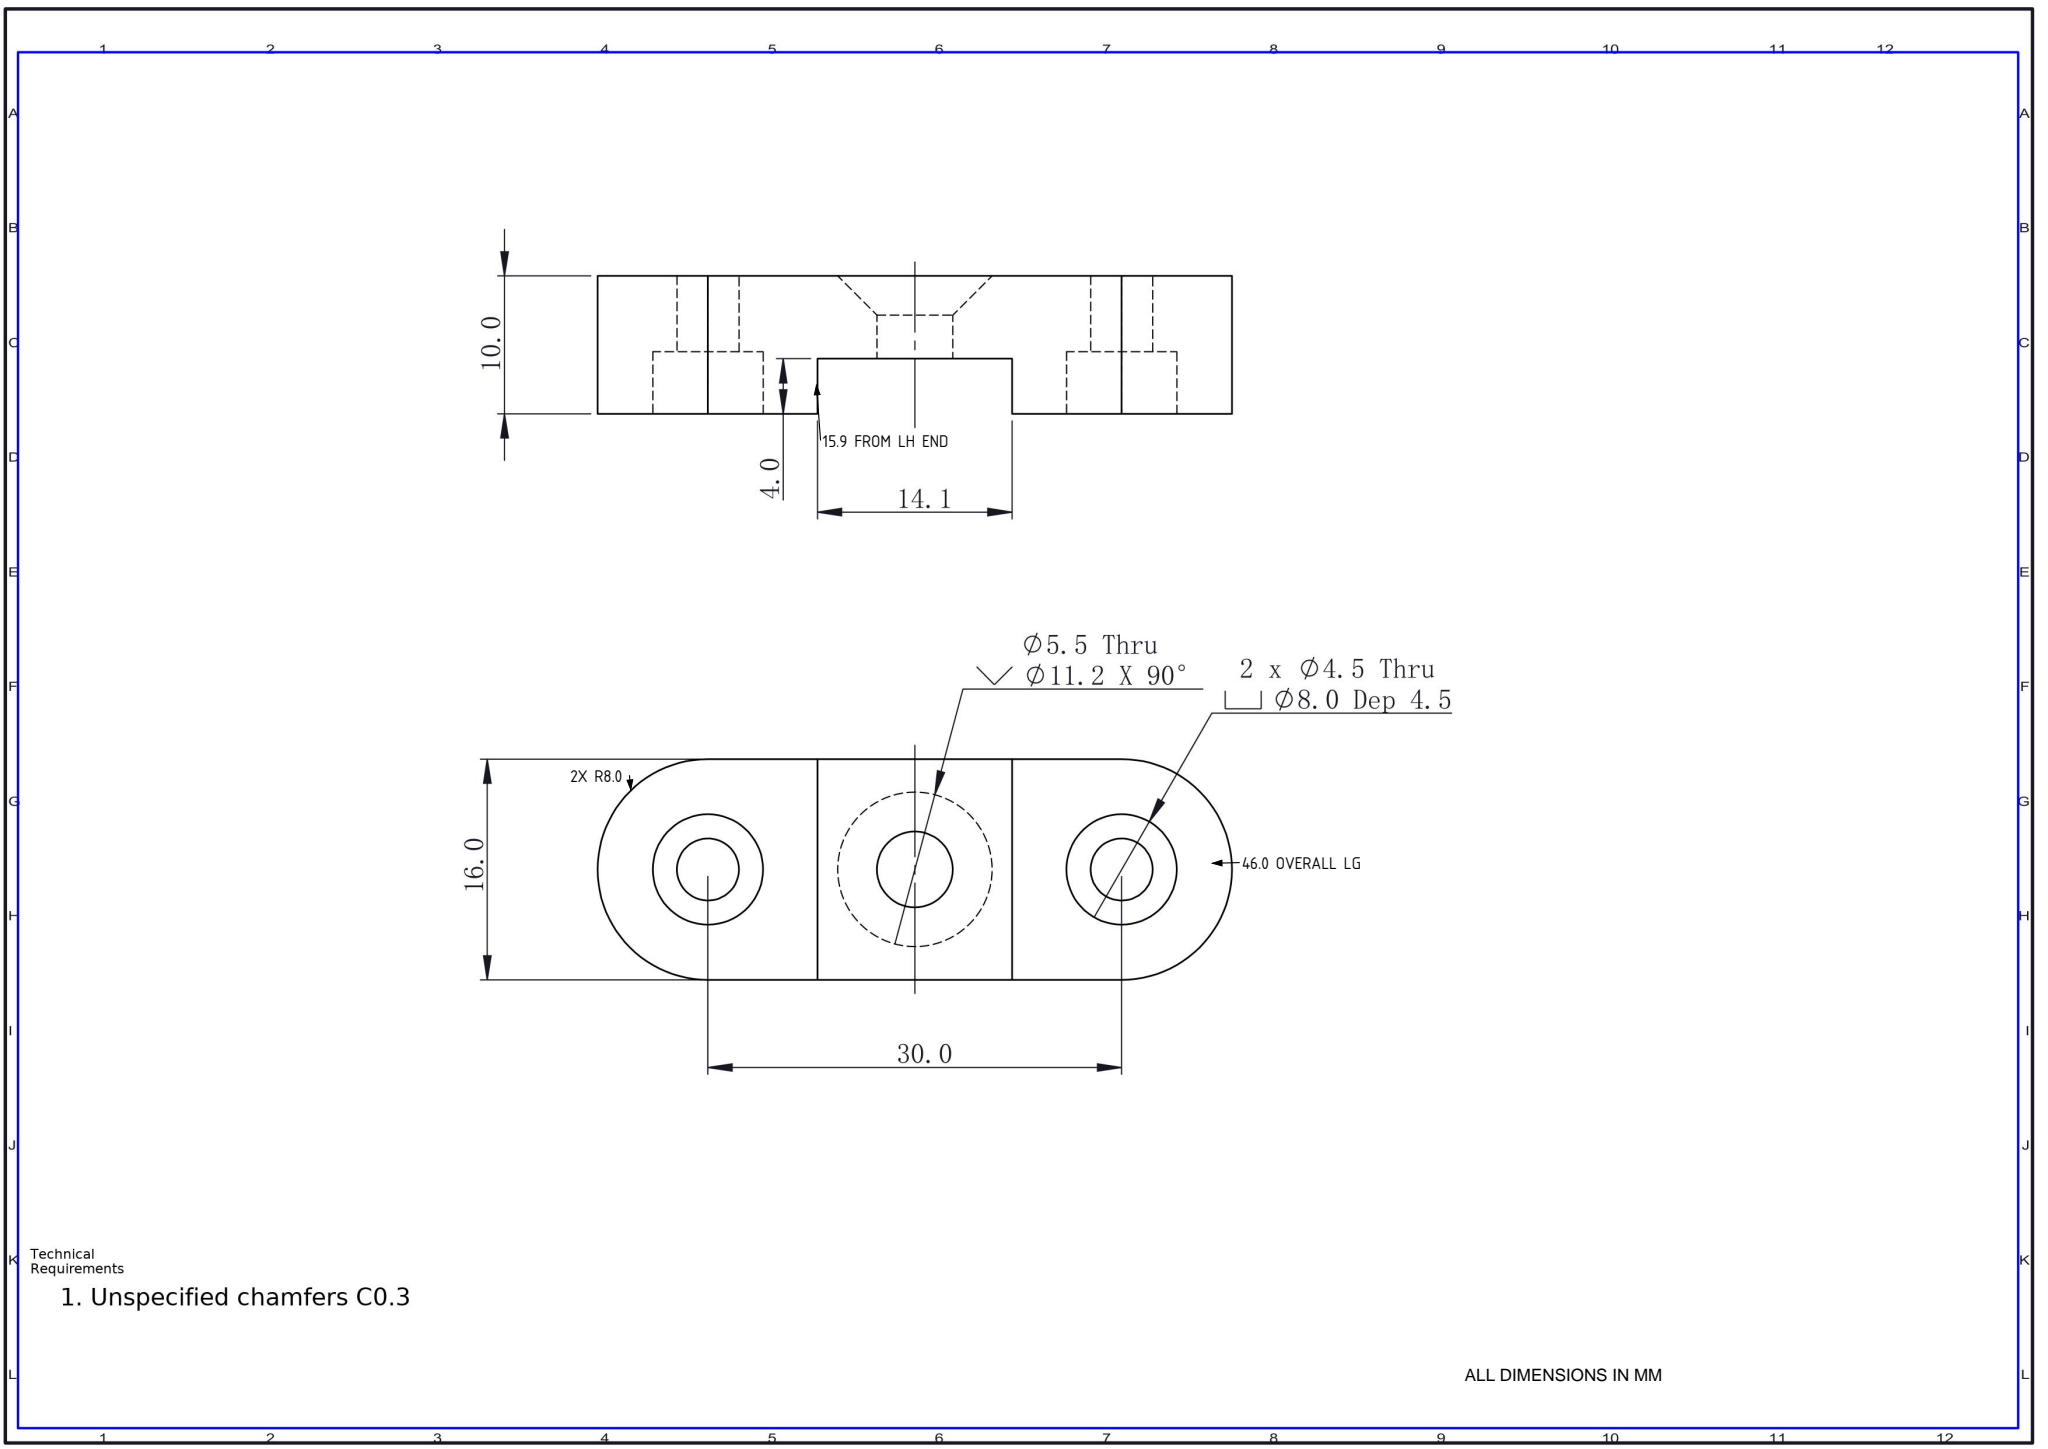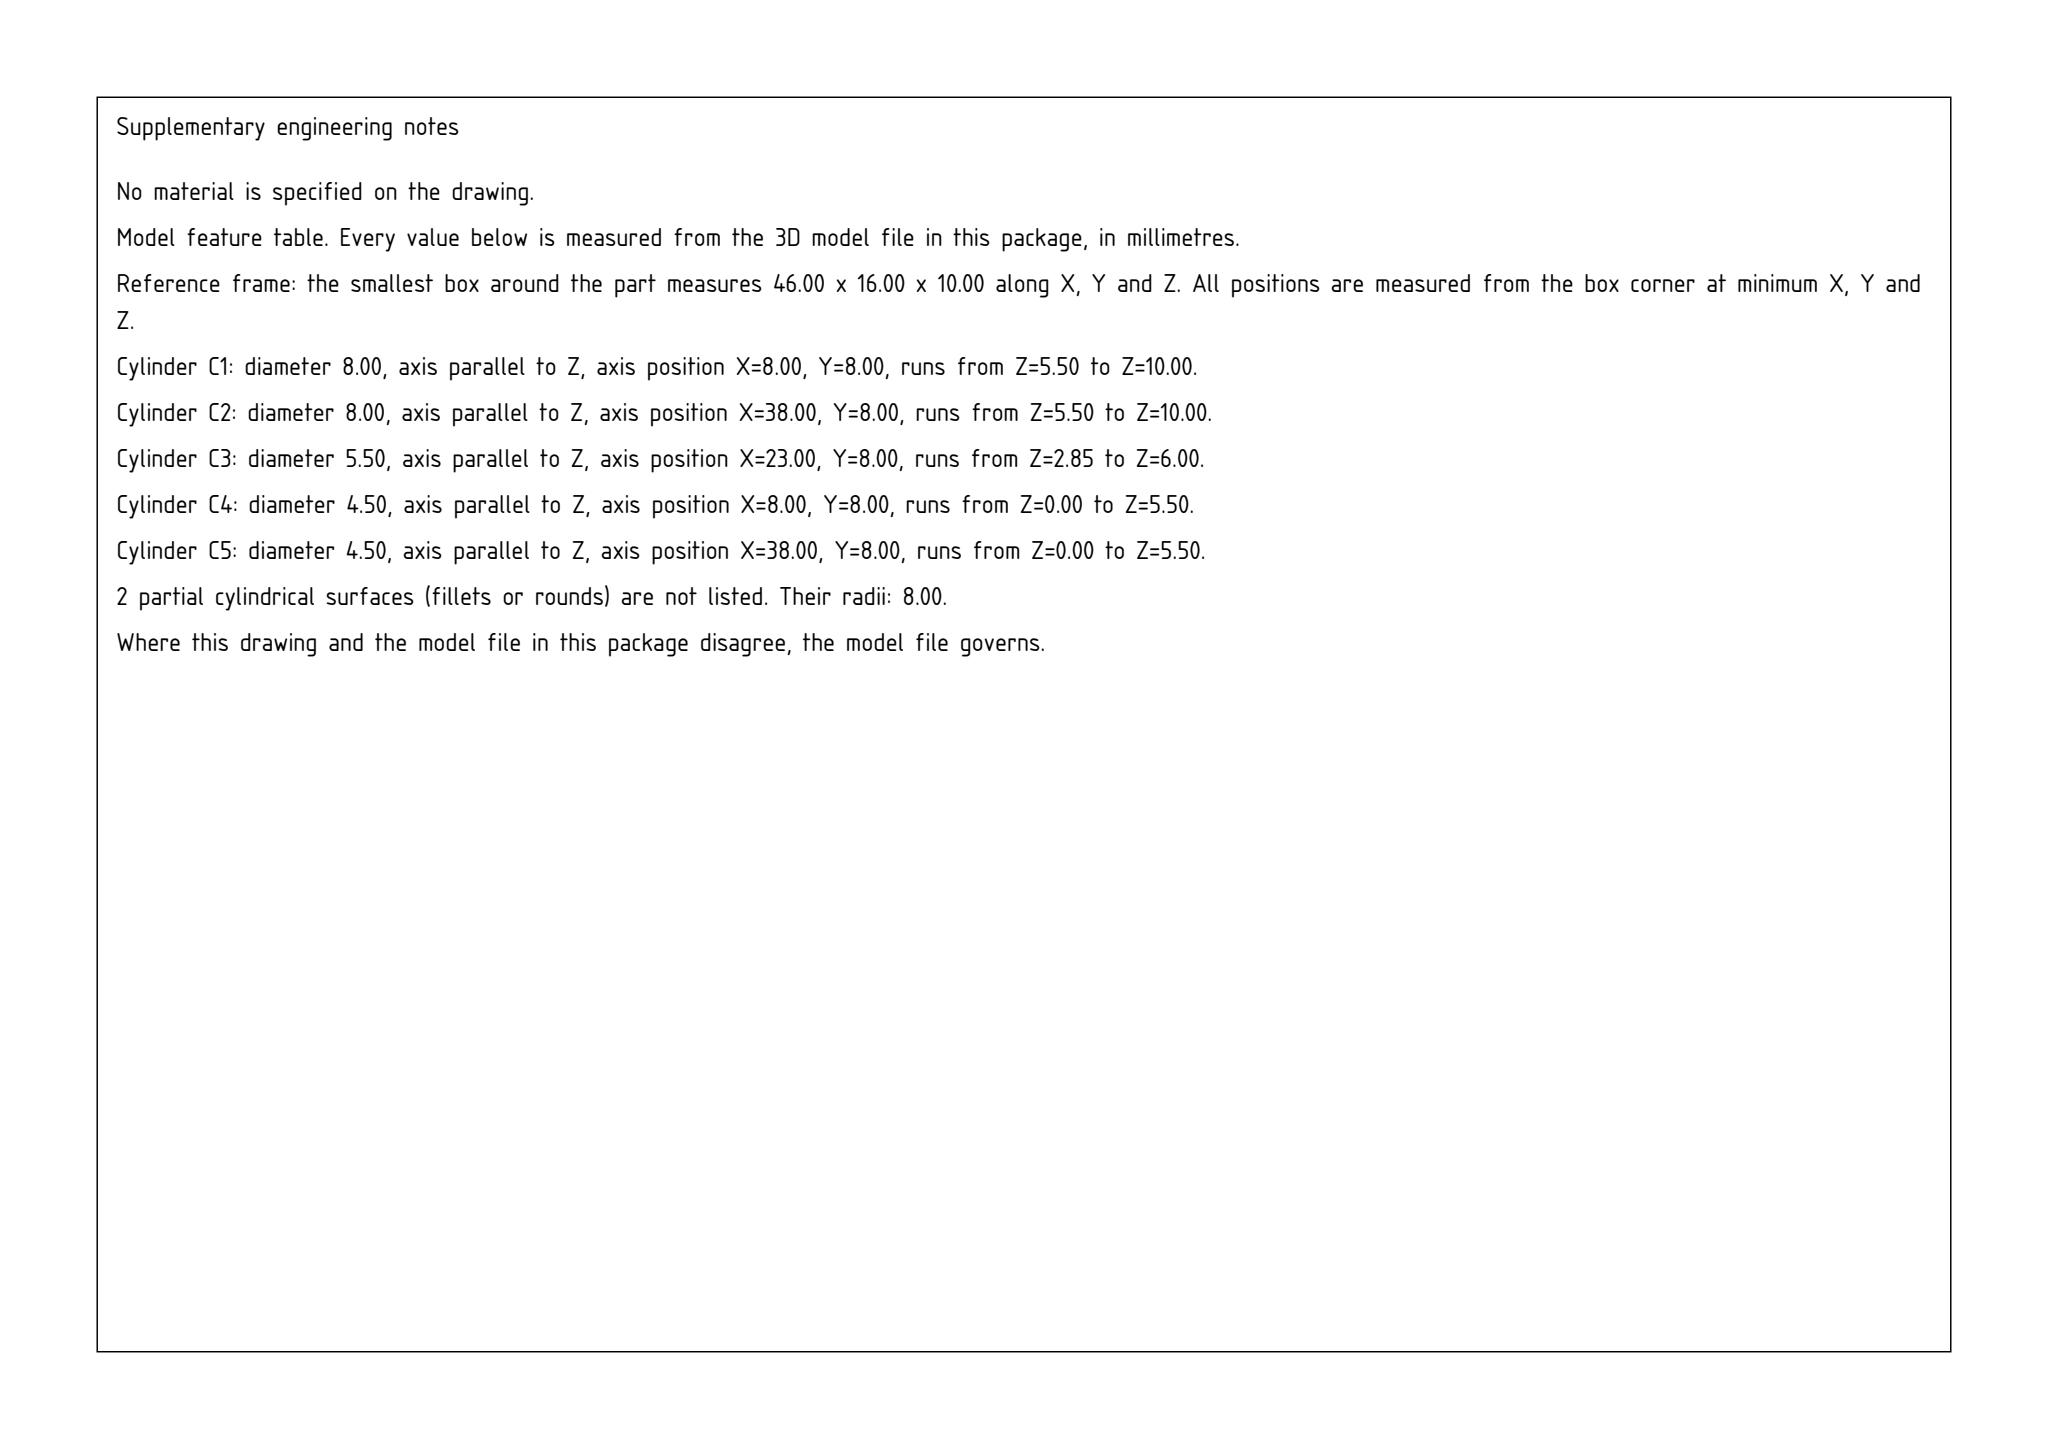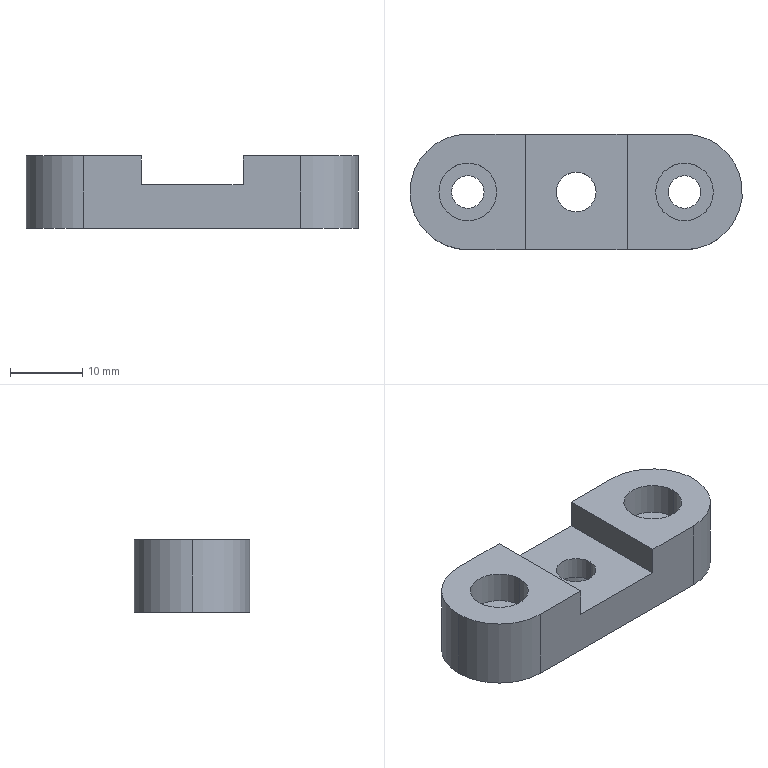Part | SolidWorks | mm | 1 solid | 25 faces | box 46 x 16 x 10 mm | volume 5044 mm3 | cylinder 13 | plane 10 | cone 2 | commonest cylinder face diameters 8 x4 4.5 x4 16 x3 5.5 x2
Drawing notes:
OVERALL LG 46.0; Ø4.5 HOLE CL 8.0 FROM EACH END | from the solid: bbox_xyz x=46.0; Ø4.5 holes at x=8.0 and x=38.0 (46-38=8.0)
2X R8.0 ENDS, CTRS ON Ø4.5 HOLE CL (16.0 WIDE) | from the solid: convex arcs dia 16.0 (R8.0), 180 deg, at [8.0,8.0] and [38.0,8.0]
STEP 14.1 WIDE X 4.0 DP: LH WALL 15.9 FROM LH END | from the solid: x-planes at 15.9 and 30.0 (z 6.0-10.0); floor z=5.?/6.0 vs top z=10.0
build123d program:
from build123d import *

# Parameters (mm, degrees)
BOSS_EXTRUDE1_DEPTH                                  = 10
M4_HEX_SOCKET_HEAD_CAP_SCREW_CBORE1_D                = 4.5
M4_HEX_SOCKET_HEAD_CAP_SCREW_CBORE1_CBORE_D          = 8
M4_HEX_SOCKET_HEAD_CAP_SCREW_CBORE1_CBORE_DEPTH      = 4.5
SKETCH4_W                                            = 14.1
SKETCH4_H                                            = 16
CUT_EXTRUDE1_DEPTH                                   = 4
COUNTERSUNK_HOLE_1_FOR_M5_HEX_SOCKET_COU_D           = 5.5
COUNTERSUNK_HOLE_1_FOR_M5_HEX_SOCKET_COU_CSINK_D     = 11.2
COUNTERSUNK_HOLE_1_FOR_M5_HEX_SOCKET_COU_CSINK_ANGLE = 90


with BuildPart() as part:
    # Sketch1 → Boss-Extrude1 (new body)
    with BuildSketch(Plane.XY):
        with BuildLine():
            Line((0, 8), (30, 8))
            ThreePointArc((30, 8), (38, 0), (30, -8))
            Line((30, -8), (0, -8))
            ThreePointArc((0, -8), (-8, 0), (0, 8))
        make_face()
    extrude(amount=BOSS_EXTRUDE1_DEPTH)

    # M4 Hex Socket Head Cap Screw CBORE1 (through all)
    with Locations(Plane.XY.offset(10)):
        with Locations((0, 0), (30, 0)):
            CounterBoreHole(M4_HEX_SOCKET_HEAD_CAP_SCREW_CBORE1_D / 2, M4_HEX_SOCKET_HEAD_CAP_SCREW_CBORE1_CBORE_D / 2, M4_HEX_SOCKET_HEAD_CAP_SCREW_CBORE1_CBORE_DEPTH)

    # Sketch4 → Cut-Extrude1 (cut)
    with BuildSketch(Plane.XY.offset(10)):
        with Locations((15, 0)):
            Rectangle(SKETCH4_W, SKETCH4_H)
    extrude(amount=-CUT_EXTRUDE1_DEPTH, mode=Mode.SUBTRACT)

    # Countersunk hole 1 for M5 hex socket cou (through all)
    with Locations(Plane(origin=(0, 0, 0), x_dir=(-1, 0, 0), z_dir=(0, 0, -1))):
        with Locations((-15, 0)):
            CounterSinkHole(COUNTERSUNK_HOLE_1_FOR_M5_HEX_SOCKET_COU_D / 2, COUNTERSUNK_HOLE_1_FOR_M5_HEX_SOCKET_COU_CSINK_D / 2, counter_sink_angle=COUNTERSUNK_HOLE_1_FOR_M5_HEX_SOCKET_COU_CSINK_ANGLE)


solid = part.part
STEP:
#1=CARTESIAN_POINT('',(17.75,0.,2.85));
#2=VERTEX_POINT('',#1);
#3=CARTESIAN_POINT('',(12.25,0.,2.85));
#4=VERTEX_POINT('',#3);
#5=CARTESIAN_POINT('',(15.,0.,2.85));
#6=DIRECTION('',(0.,0.,-1.));
#7=DIRECTION('',(-1.,0.,0.));
#8=AXIS2_PLACEMENT_3D('',#5,#6,#7);
#9=CIRCLE('',#8,2.75);
#10=EDGE_CURVE('',#2,#4,#9,.T.);
#11=ORIENTED_EDGE('',*,*,#10,.F.);
#12=CARTESIAN_POINT('',(20.6,0.,-0.));
#13=VERTEX_POINT('',#12);
#14=CARTESIAN_POINT('',(20.6,0.,-0.));
#15=DIRECTION('',(0.7071,0.,-0.7071));
#16=VECTOR('',#15,1000.);
#17=LINE('',#14,#16);
#18=EDGE_CURVE('',#2,#13,#17,.T.);
#19=ORIENTED_EDGE('',*,*,#18,.T.);
#20=CARTESIAN_POINT('',(9.4,0.,-0.));
#21=VERTEX_POINT('',#20);
#22=CARTESIAN_POINT('',(15.,0.,-0.));
#23=DIRECTION('',(0.,0.,-1.));
#24=DIRECTION('',(-1.,0.,0.));
#25=AXIS2_PLACEMENT_3D('',#22,#23,#24);
#26=CIRCLE('',#25,5.6);
#27=EDGE_CURVE('',#13,#21,#26,.T.);
#28=ORIENTED_EDGE('',*,*,#27,.T.);
#29=CARTESIAN_POINT('',(9.4,0.,-0.));
#30=DIRECTION('',(-0.7071,0.,-0.7071));
#31=VECTOR('',#30,1000.);
#32=LINE('',#29,#31);
#33=EDGE_CURVE('',#4,#21,#32,.T.);
#34=ORIENTED_EDGE('',*,*,#33,.F.);
#35=EDGE_LOOP('',(#11,#19,#28,#34));
#36=FACE_OUTER_BOUND('',#35,.T.);
#37=CARTESIAN_POINT('',(15.,0.,-0.));
#38=DIRECTION('',(0.,0.,-1.));
#39=DIRECTION('',(-1.,0.,0.));
#40=AXIS2_PLACEMENT_3D('',#37,#38,#39);
#41=CONICAL_SURFACE('',#40,5.6,0.7854);
#42=ADVANCED_FACE('',(#36),#41,.F.);
#43=CARTESIAN_POINT('',(12.25,0.,6.));
#44=VERTEX_POINT('',#43);
#45=CARTESIAN_POINT('',(17.75,0.,6.));
#46=VERTEX_POINT('',#45);
#47=CARTESIAN_POINT('',(15.,0.,6.));
#48=DIRECTION('',(0.,0.,1.));
#49=DIRECTION('',(1.,0.,0.));
#50=AXIS2_PLACEMENT_3D('',#47,#48,#49);
#51=CIRCLE('',#50,2.75);
#52=EDGE_CURVE('',#44,#46,#51,.T.);
#53=ORIENTED_EDGE('',*,*,#52,.T.);
#54=CARTESIAN_POINT('',(17.75,0.,0.));
#55=DIRECTION('',(0.,0.,-1.));
#56=VECTOR('',#55,1000.);
#57=LINE('',#54,#56);
#58=EDGE_CURVE('',#46,#2,#57,.T.);
#59=ORIENTED_EDGE('',*,*,#58,.T.);
#60=ORIENTED_EDGE('',*,*,#10,.T.);
#61=CARTESIAN_POINT('',(12.25,0.,0.));
#62=DIRECTION('',(0.,0.,-1.));
#63=VECTOR('',#62,1000.);
#64=LINE('',#61,#63);
#65=EDGE_CURVE('',#44,#4,#64,.T.);
#66=ORIENTED_EDGE('',*,*,#65,.F.);
#67=EDGE_LOOP('',(#53,#59,#60,#66));
#68=FACE_OUTER_BOUND('',#67,.T.);
#69=CARTESIAN_POINT('',(15.,0.,0.));
#70=DIRECTION('',(0.,0.,-1.));
#71=DIRECTION('',(-1.,0.,0.));
#72=AXIS2_PLACEMENT_3D('',#69,#70,#71);
#73=CYLINDRICAL_SURFACE('',#72,2.75);
#74=ADVANCED_FACE('',(#68),#73,.F.);
#75=CARTESIAN_POINT('',(-4.,0.,5.5));
#76=VERTEX_POINT('',#75);
#77=CARTESIAN_POINT('',(4.,0.,5.5));
#78=VERTEX_POINT('',#77);
#79=CARTESIAN_POINT('',(0.,0.,5.5));
#80=DIRECTION('',(0.,0.,1.));
#81=DIRECTION('',(1.,0.,0.));
#82=AXIS2_PLACEMENT_3D('',#79,#80,#81);
#83=CIRCLE('',#82,4.);
#84=EDGE_CURVE('',#76,#78,#83,.T.);
#85=ORIENTED_EDGE('',*,*,#84,.F.);
#86=CARTESIAN_POINT('',(-4.,0.,10.));
#87=VERTEX_POINT('',#86);
#88=CARTESIAN_POINT('',(-4.,0.,10.));
#89=DIRECTION('',(0.,0.,1.));
#90=VECTOR('',#89,1000.);
#91=LINE('',#88,#90);
#92=EDGE_CURVE('',#76,#87,#91,.T.);
#93=ORIENTED_EDGE('',*,*,#92,.T.);
#94=CARTESIAN_POINT('',(4.,0.,10.));
#95=VERTEX_POINT('',#94);
#96=CARTESIAN_POINT('',(0.,0.,10.));
#97=DIRECTION('',(0.,0.,1.));
#98=DIRECTION('',(1.,0.,0.));
#99=AXIS2_PLACEMENT_3D('',#96,#97,#98);
#100=CIRCLE('',#99,4.);
#101=EDGE_CURVE('',#87,#95,#100,.T.);
#102=ORIENTED_EDGE('',*,*,#101,.T.);
#103=CARTESIAN_POINT('',(4.,0.,10.));
#104=DIRECTION('',(0.,0.,1.));
#105=VECTOR('',#104,1000.);
#106=LINE('',#103,#105);
#107=EDGE_CURVE('',#78,#95,#106,.T.);
#108=ORIENTED_EDGE('',*,*,#107,.F.);
#109=EDGE_LOOP('',(#85,#93,#102,#108));
#110=FACE_OUTER_BOUND('',#109,.T.);
#111=CARTESIAN_POINT('',(0.,0.,10.));
#112=DIRECTION('',(0.,0.,1.));
#113=DIRECTION('',(1.,0.,0.));
#114=AXIS2_PLACEMENT_3D('',#111,#112,#113);
#115=CYLINDRICAL_SURFACE('',#114,4.);
#116=ADVANCED_FACE('',(#110),#115,.F.);
#117=CARTESIAN_POINT('',(-2.25,0.,0.));
#118=VERTEX_POINT('',#117);
#119=CARTESIAN_POINT('',(2.25,0.,0.));
#120=VERTEX_POINT('',#119);
#121=CARTESIAN_POINT('',(0.,0.,0.));
#122=DIRECTION('',(0.,0.,1.));
#123=DIRECTION('',(1.,0.,0.));
#124=AXIS2_PLACEMENT_3D('',#121,#122,#123);
#125=CIRCLE('',#124,2.25);
#126=EDGE_CURVE('',#118,#120,#125,.T.);
#127=ORIENTED_EDGE('',*,*,#126,.F.);
#128=CARTESIAN_POINT('',(-2.25,0.,5.5));
#129=VERTEX_POINT('',#128);
#130=CARTESIAN_POINT('',(-2.25,0.,10.));
#131=DIRECTION('',(0.,0.,1.));
#132=VECTOR('',#131,1000.);
#133=LINE('',#130,#132);
#134=EDGE_CURVE('',#118,#129,#133,.T.);
#135=ORIENTED_EDGE('',*,*,#134,.T.);
#136=CARTESIAN_POINT('',(2.25,0.,5.5));
#137=VERTEX_POINT('',#136);
#138=CARTESIAN_POINT('',(0.,0.,5.5));
#139=DIRECTION('',(0.,0.,1.));
#140=DIRECTION('',(1.,0.,0.));
#141=AXIS2_PLACEMENT_3D('',#138,#139,#140);
#142=CIRCLE('',#141,2.25);
#143=EDGE_CURVE('',#129,#137,#142,.T.);
#144=ORIENTED_EDGE('',*,*,#143,.T.);
#145=CARTESIAN_POINT('',(2.25,0.,10.));
#146=DIRECTION('',(0.,0.,1.));
#147=VECTOR('',#146,1000.);
#148=LINE('',#145,#147);
#149=EDGE_CURVE('',#120,#137,#148,.T.);
#150=ORIENTED_EDGE('',*,*,#149,.F.);
#151=EDGE_LOOP('',(#127,#135,#144,#150));
#152=FACE_OUTER_BOUND('',#151,.T.);
#153=CARTESIAN_POINT('',(0.,0.,10.));
#154=DIRECTION('',(0.,0.,1.));
#155=DIRECTION('',(1.,0.,0.));
#156=AXIS2_PLACEMENT_3D('',#153,#154,#155);
#157=CYLINDRICAL_SURFACE('',#156,2.25);
#158=ADVANCED_FACE('',(#152),#157,.F.);
#159=CARTESIAN_POINT('',(26.,0.,5.5));
#160=VERTEX_POINT('',#159);
#161=CARTESIAN_POINT('',(34.,0.,5.5));
#162=VERTEX_POINT('',#161);
#163=CARTESIAN_POINT('',(30.,0.,5.5));
#164=DIRECTION('',(0.,0.,1.));
#165=DIRECTION('',(1.,0.,0.));
#166=AXIS2_PLACEMENT_3D('',#163,#164,#165);
#167=CIRCLE('',#166,4.);
#168=EDGE_CURVE('',#160,#162,#167,.T.);
#169=ORIENTED_EDGE('',*,*,#168,.F.);
#170=CARTESIAN_POINT('',(26.,0.,10.));
#171=VERTEX_POINT('',#170);
#172=CARTESIAN_POINT('',(26.,0.,10.));
#173=DIRECTION('',(0.,0.,1.));
#174=VECTOR('',#173,1000.);
#175=LINE('',#172,#174);
#176=EDGE_CURVE('',#160,#171,#175,.T.);
#177=ORIENTED_EDGE('',*,*,#176,.T.);
#178=CARTESIAN_POINT('',(34.,0.,10.));
#179=VERTEX_POINT('',#178);
#180=CARTESIAN_POINT('',(30.,0.,10.));
#181=DIRECTION('',(0.,0.,1.));
#182=DIRECTION('',(1.,0.,0.));
#183=AXIS2_PLACEMENT_3D('',#180,#181,#182);
#184=CIRCLE('',#183,4.);
#185=EDGE_CURVE('',#171,#179,#184,.T.);
#186=ORIENTED_EDGE('',*,*,#185,.T.);
#187=CARTESIAN_POINT('',(34.,0.,10.));
#188=DIRECTION('',(0.,0.,1.));
#189=VECTOR('',#188,1000.);
#190=LINE('',#187,#189);
#191=EDGE_CURVE('',#162,#179,#190,.T.);
#192=ORIENTED_EDGE('',*,*,#191,.F.);
#193=EDGE_LOOP('',(#169,#177,#186,#192));
#194=FACE_OUTER_BOUND('',#193,.T.);
#195=CARTESIAN_POINT('',(30.,0.,10.));
#196=DIRECTION('',(0.,0.,1.));
#197=DIRECTION('',(1.,0.,0.));
#198=AXIS2_PLACEMENT_3D('',#195,#196,#197);
#199=CYLINDRICAL_SURFACE('',#198,4.);
#200=ADVANCED_FACE('',(#194),#199,.F.);
#201=CARTESIAN_POINT('',(27.75,0.,0.));
#202=VERTEX_POINT('',#201);
#203=CARTESIAN_POINT('',(32.25,0.,0.));
#204=VERTEX_POINT('',#203);
#205=CARTESIAN_POINT('',(30.,0.,0.));
#206=DIRECTION('',(0.,0.,1.));
#207=DIRECTION('',(1.,0.,0.));
#208=AXIS2_PLACEMENT_3D('',#205,#206,#207);
#209=CIRCLE('',#208,2.25);
#210=EDGE_CURVE('',#202,#204,#209,.T.);
#211=ORIENTED_EDGE('',*,*,#210,.F.);
#212=CARTESIAN_POINT('',(27.75,0.,5.5));
#213=VERTEX_POINT('',#212);
#214=CARTESIAN_POINT('',(27.75,0.,10.));
#215=DIRECTION('',(0.,0.,1.));
#216=VECTOR('',#215,1000.);
#217=LINE('',#214,#216);
#218=EDGE_CURVE('',#202,#213,#217,.T.);
#219=ORIENTED_EDGE('',*,*,#218,.T.);
#220=CARTESIAN_POINT('',(32.25,0.,5.5));
#221=VERTEX_POINT('',#220);
#222=CARTESIAN_POINT('',(30.,0.,5.5));
#223=DIRECTION('',(0.,0.,1.));
#224=DIRECTION('',(1.,0.,0.));
#225=AXIS2_PLACEMENT_3D('',#222,#223,#224);
#226=CIRCLE('',#225,2.25);
#227=EDGE_CURVE('',#213,#221,#226,.T.);
#228=ORIENTED_EDGE('',*,*,#227,.T.);
#229=CARTESIAN_POINT('',(32.25,0.,10.));
#230=DIRECTION('',(0.,0.,1.));
#231=VECTOR('',#230,1000.);
#232=LINE('',#229,#231);
#233=EDGE_CURVE('',#204,#221,#232,.T.);
#234=ORIENTED_EDGE('',*,*,#233,.F.);
#235=EDGE_LOOP('',(#211,#219,#228,#234));
#236=FACE_OUTER_BOUND('',#235,.T.);
#237=CARTESIAN_POINT('',(30.,0.,10.));
#238=DIRECTION('',(0.,0.,1.));
#239=DIRECTION('',(1.,0.,0.));
#240=AXIS2_PLACEMENT_3D('',#237,#238,#239);
#241=CYLINDRICAL_SURFACE('',#240,2.25);
#242=ADVANCED_FACE('',(#236),#241,.F.);
#243=CARTESIAN_POINT('',(-8.,0.,10.));
#244=VERTEX_POINT('',#243);
#245=CARTESIAN_POINT('',(0.,-8.,10.));
#246=VERTEX_POINT('',#245);
#247=CARTESIAN_POINT('',(0.,0.,10.));
#248=DIRECTION('',(0.,0.,1.));
#249=DIRECTION('',(1.,0.,0.));
#250=AXIS2_PLACEMENT_3D('',#247,#248,#249);
#251=CIRCLE('',#250,8.);
#252=EDGE_CURVE('',#244,#246,#251,.T.);
#253=ORIENTED_EDGE('',*,*,#252,.F.);
#254=CARTESIAN_POINT('',(-8.,0.,0.));
#255=VERTEX_POINT('',#254);
#256=CARTESIAN_POINT('',(-8.,0.,10.));
#257=DIRECTION('',(0.,0.,-1.));
#258=VECTOR('',#257,1000.);
#259=LINE('',#256,#258);
#260=EDGE_CURVE('',#244,#255,#259,.T.);
#261=ORIENTED_EDGE('',*,*,#260,.T.);
#262=CARTESIAN_POINT('',(0.,-8.,0.));
#263=VERTEX_POINT('',#262);
#264=CARTESIAN_POINT('',(0.,0.,0.));
#265=DIRECTION('',(0.,0.,1.));
#266=DIRECTION('',(1.,0.,0.));
#267=AXIS2_PLACEMENT_3D('',#264,#265,#266);
#268=CIRCLE('',#267,8.);
#269=EDGE_CURVE('',#255,#263,#268,.T.);
#270=ORIENTED_EDGE('',*,*,#269,.T.);
#271=CARTESIAN_POINT('',(0.,-8.,10.));
#272=DIRECTION('',(0.,0.,-1.));
#273=VECTOR('',#272,1000.);
#274=LINE('',#271,#273);
#275=EDGE_CURVE('',#246,#263,#274,.T.);
#276=ORIENTED_EDGE('',*,*,#275,.F.);
#277=EDGE_LOOP('',(#253,#261,#270,#276));
#278=FACE_OUTER_BOUND('',#277,.T.);
#279=CARTESIAN_POINT('',(0.,0.,10.));
#280=DIRECTION('',(0.,0.,-1.));
#281=DIRECTION('',(-1.,0.,0.));
#282=AXIS2_PLACEMENT_3D('',#279,#280,#281);
#283=CYLINDRICAL_SURFACE('',#282,8.);
#284=ADVANCED_FACE('',(#278),#283,.T.);
#285=CARTESIAN_POINT('',(7.95,8.,10.));
#286=VERTEX_POINT('',#285);
#287=CARTESIAN_POINT('',(7.95,-8.,10.));
#288=VERTEX_POINT('',#287);
#289=CARTESIAN_POINT('',(7.95,8.,10.));
#290=DIRECTION('',(0.,-1.,0.));
#291=VECTOR('',#290,1000.);
#292=LINE('',#289,#291);
#293=EDGE_CURVE('',#286,#288,#292,.T.);
#294=ORIENTED_EDGE('',*,*,#293,.F.);
#295=CARTESIAN_POINT('',(0.,8.,10.));
#296=VERTEX_POINT('',#295);
#297=CARTESIAN_POINT('',(0.,8.,10.));
#298=DIRECTION('',(-1.,0.,0.));
#299=VECTOR('',#298,1000.);
#300=LINE('',#297,#299);
#301=EDGE_CURVE('',#286,#296,#300,.T.);
#302=ORIENTED_EDGE('',*,*,#301,.T.);
#303=CARTESIAN_POINT('',(0.,0.,10.));
#304=DIRECTION('',(0.,0.,1.));
#305=DIRECTION('',(1.,0.,0.));
#306=AXIS2_PLACEMENT_3D('',#303,#304,#305);
#307=CIRCLE('',#306,8.);
#308=EDGE_CURVE('',#296,#244,#307,.T.);
#309=ORIENTED_EDGE('',*,*,#308,.T.);
#310=ORIENTED_EDGE('',*,*,#252,.T.);
#311=CARTESIAN_POINT('',(0.,-8.,10.));
#312=DIRECTION('',(1.,0.,0.));
#313=VECTOR('',#312,1000.);
#314=LINE('',#311,#313);
#315=EDGE_CURVE('',#246,#288,#314,.T.);
#316=ORIENTED_EDGE('',*,*,#315,.T.);
#317=EDGE_LOOP('',(#294,#302,#309,#310,#316));
#318=FACE_OUTER_BOUND('',#317,.T.);
#319=CARTESIAN_POINT('',(0.,0.,10.));
#320=DIRECTION('',(0.,0.,1.));
#321=DIRECTION('',(1.,0.,0.));
#322=AXIS2_PLACEMENT_3D('',#319,#320,#321);
#323=CIRCLE('',#322,4.);
#324=EDGE_CURVE('',#95,#87,#323,.T.);
#325=ORIENTED_EDGE('',*,*,#324,.F.);
#326=ORIENTED_EDGE('',*,*,#101,.F.);
#327=EDGE_LOOP('',(#325,#326));
#328=FACE_BOUND('',#327,.T.);
#329=CARTESIAN_POINT('',(0.,0.,10.));
#330=DIRECTION('',(0.,0.,1.));
#331=DIRECTION('',(1.,0.,0.));
#332=AXIS2_PLACEMENT_3D('',#329,#330,#331);
#333=PLANE('',#332);
#334=ADVANCED_FACE('',(#318,#328),#333,.T.);
#335=ORIENTED_EDGE('',*,*,#260,.F.);
#336=ORIENTED_EDGE('',*,*,#308,.F.);
#337=CARTESIAN_POINT('',(0.,8.,0.));
#338=VERTEX_POINT('',#337);
#339=CARTESIAN_POINT('',(0.,8.,10.));
#340=DIRECTION('',(0.,0.,-1.));
#341=VECTOR('',#340,1000.);
#342=LINE('',#339,#341);
#343=EDGE_CURVE('',#296,#338,#342,.T.);
#344=ORIENTED_EDGE('',*,*,#343,.T.);
#345=CARTESIAN_POINT('',(0.,0.,0.));
#346=DIRECTION('',(0.,0.,1.));
#347=DIRECTION('',(1.,0.,0.));
#348=AXIS2_PLACEMENT_3D('',#345,#346,#347);
#349=CIRCLE('',#348,8.);
#350=EDGE_CURVE('',#338,#255,#349,.T.);
#351=ORIENTED_EDGE('',*,*,#350,.T.);
#352=EDGE_LOOP('',(#335,#336,#344,#351));
#353=FACE_OUTER_BOUND('',#352,.T.);
#354=CARTESIAN_POINT('',(0.,0.,10.));
#355=DIRECTION('',(0.,0.,-1.));
#356=DIRECTION('',(-1.,0.,0.));
#357=AXIS2_PLACEMENT_3D('',#354,#355,#356);
#358=CYLINDRICAL_SURFACE('',#357,8.);
#359=ADVANCED_FACE('',(#353),#358,.T.);
#360=CARTESIAN_POINT('',(7.95,-8.,6.));
#361=VERTEX_POINT('',#360);
#362=CARTESIAN_POINT('',(22.05,-8.,6.));
#363=VERTEX_POINT('',#362);
#364=CARTESIAN_POINT('',(7.95,-8.,6.));
#365=DIRECTION('',(1.,0.,0.));
#366=VECTOR('',#365,1000.);
#367=LINE('',#364,#366);
#368=EDGE_CURVE('',#361,#363,#367,.T.);
#369=ORIENTED_EDGE('',*,*,#368,.F.);
#370=CARTESIAN_POINT('',(7.95,-8.,6.));
#371=DIRECTION('',(0.,0.,1.));
#372=VECTOR('',#371,1000.);
#373=LINE('',#370,#372);
#374=EDGE_CURVE('',#361,#288,#373,.T.);
#375=ORIENTED_EDGE('',*,*,#374,.T.);
#376=ORIENTED_EDGE('',*,*,#315,.F.);
#377=ORIENTED_EDGE('',*,*,#275,.T.);
#378=CARTESIAN_POINT('',(30.,-8.,0.));
#379=VERTEX_POINT('',#378);
#380=CARTESIAN_POINT('',(0.,-8.,0.));
#381=DIRECTION('',(1.,0.,0.));
#382=VECTOR('',#381,1000.);
#383=LINE('',#380,#382);
#384=EDGE_CURVE('',#263,#379,#383,.T.);
#385=ORIENTED_EDGE('',*,*,#384,.T.);
#386=CARTESIAN_POINT('',(30.,-8.,10.));
#387=VERTEX_POINT('',#386);
#388=CARTESIAN_POINT('',(30.,-8.,10.));
#389=DIRECTION('',(0.,0.,-1.));
#390=VECTOR('',#389,1000.);
#391=LINE('',#388,#390);
#392=EDGE_CURVE('',#387,#379,#391,.T.);
#393=ORIENTED_EDGE('',*,*,#392,.F.);
#394=CARTESIAN_POINT('',(22.05,-8.,10.));
#395=VERTEX_POINT('',#394);
#396=CARTESIAN_POINT('',(0.,-8.,10.));
#397=DIRECTION('',(1.,0.,0.));
#398=VECTOR('',#397,1000.);
#399=LINE('',#396,#398);
#400=EDGE_CURVE('',#395,#387,#399,.T.);
#401=ORIENTED_EDGE('',*,*,#400,.F.);
#402=CARTESIAN_POINT('',(22.05,-8.,6.));
#403=DIRECTION('',(0.,0.,1.));
#404=VECTOR('',#403,1000.);
#405=LINE('',#402,#404);
#406=EDGE_CURVE('',#363,#395,#405,.T.);
#407=ORIENTED_EDGE('',*,*,#406,.F.);
#408=EDGE_LOOP('',(#369,#375,#376,#377,#385,#393,#401,#407));
#409=FACE_OUTER_BOUND('',#408,.T.);
#410=CARTESIAN_POINT('',(0.,-8.,10.));
#411=DIRECTION('',(0.,1.,0.));
#412=DIRECTION('',(0.,0.,1.));
#413=AXIS2_PLACEMENT_3D('',#410,#411,#412);
#414=PLANE('',#413);
#415=ADVANCED_FACE('',(#409),#414,.F.);
#416=CARTESIAN_POINT('',(30.,8.,0.));
#417=VERTEX_POINT('',#416);
#418=CARTESIAN_POINT('',(30.,0.,0.));
#419=DIRECTION('',(0.,0.,1.));
#420=DIRECTION('',(1.,0.,0.));
#421=AXIS2_PLACEMENT_3D('',#418,#419,#420);
#422=CIRCLE('',#421,8.);
#423=EDGE_CURVE('',#379,#417,#422,.T.);
#424=ORIENTED_EDGE('',*,*,#423,.T.);
#425=CARTESIAN_POINT('',(30.,8.,10.));
#426=VERTEX_POINT('',#425);
#427=CARTESIAN_POINT('',(30.,8.,10.));
#428=DIRECTION('',(0.,0.,-1.));
#429=VECTOR('',#428,1000.);
#430=LINE('',#427,#429);
#431=EDGE_CURVE('',#426,#417,#430,.T.);
#432=ORIENTED_EDGE('',*,*,#431,.F.);
#433=CARTESIAN_POINT('',(30.,0.,10.));
#434=DIRECTION('',(0.,0.,1.));
#435=DIRECTION('',(1.,0.,0.));
#436=AXIS2_PLACEMENT_3D('',#433,#434,#435);
#437=CIRCLE('',#436,8.);
#438=EDGE_CURVE('',#387,#426,#437,.T.);
#439=ORIENTED_EDGE('',*,*,#438,.F.);
#440=ORIENTED_EDGE('',*,*,#392,.T.);
#441=EDGE_LOOP('',(#424,#432,#439,#440));
#442=FACE_OUTER_BOUND('',#441,.T.);
#443=CARTESIAN_POINT('',(30.,0.,10.));
#444=DIRECTION('',(0.,0.,-1.));
#445=DIRECTION('',(-1.,0.,0.));
#446=AXIS2_PLACEMENT_3D('',#443,#444,#445);
#447=CYLINDRICAL_SURFACE('',#446,8.);
#448=ADVANCED_FACE('',(#442),#447,.T.);
#449=ORIENTED_EDGE('',*,*,#301,.F.);
#450=CARTESIAN_POINT('',(7.95,8.,6.));
#451=VERTEX_POINT('',#450);
#452=CARTESIAN_POINT('',(7.95,8.,6.));
#453=DIRECTION('',(0.,0.,1.));
#454=VECTOR('',#453,1000.);
#455=LINE('',#452,#454);
#456=EDGE_CURVE('',#451,#286,#455,.T.);
#457=ORIENTED_EDGE('',*,*,#456,.F.);
#458=CARTESIAN_POINT('',(22.05,8.,6.));
#459=VERTEX_POINT('',#458);
#460=CARTESIAN_POINT('',(7.95,8.,6.));
#461=DIRECTION('',(-1.,-0.,0.));
#462=VECTOR('',#461,1000.);
#463=LINE('',#460,#462);
#464=EDGE_CURVE('',#459,#451,#463,.T.);
#465=ORIENTED_EDGE('',*,*,#464,.F.);
#466=CARTESIAN_POINT('',(22.05,8.,10.));
#467=VERTEX_POINT('',#466);
#468=CARTESIAN_POINT('',(22.05,8.,6.));
#469=DIRECTION('',(0.,0.,1.));
#470=VECTOR('',#469,1000.);
#471=LINE('',#468,#470);
#472=EDGE_CURVE('',#459,#467,#471,.T.);
#473=ORIENTED_EDGE('',*,*,#472,.T.);
#474=CARTESIAN_POINT('',(0.,8.,10.));
#475=DIRECTION('',(-1.,0.,0.));
#476=VECTOR('',#475,1000.);
#477=LINE('',#474,#476);
#478=EDGE_CURVE('',#426,#467,#477,.T.);
#479=ORIENTED_EDGE('',*,*,#478,.F.);
#480=ORIENTED_EDGE('',*,*,#431,.T.);
#481=CARTESIAN_POINT('',(0.,8.,0.));
#482=DIRECTION('',(-1.,0.,0.));
#483=VECTOR('',#482,1000.);
#484=LINE('',#481,#483);
#485=EDGE_CURVE('',#417,#338,#484,.T.);
#486=ORIENTED_EDGE('',*,*,#485,.T.);
#487=ORIENTED_EDGE('',*,*,#343,.F.);
#488=EDGE_LOOP('',(#449,#457,#465,#473,#479,#480,#486,#487));
#489=FACE_OUTER_BOUND('',#488,.T.);
#490=CARTESIAN_POINT('',(0.,8.,10.));
#491=DIRECTION('',(0.,-1.,0.));
#492=DIRECTION('',(0.,0.,-1.));
#493=AXIS2_PLACEMENT_3D('',#490,#491,#492);
#494=PLANE('',#493);
#495=ADVANCED_FACE('',(#489),#494,.F.);
#496=CARTESIAN_POINT('',(22.05,8.,10.));
#497=DIRECTION('',(0.,1.,0.));
#498=VECTOR('',#497,1000.);
#499=LINE('',#496,#498);
#500=EDGE_CURVE('',#395,#467,#499,.T.);
#501=ORIENTED_EDGE('',*,*,#500,.F.);
#502=ORIENTED_EDGE('',*,*,#400,.T.);
#503=ORIENTED_EDGE('',*,*,#438,.T.);
#504=ORIENTED_EDGE('',*,*,#478,.T.);
#505=EDGE_LOOP('',(#501,#502,#503,#504));
#506=FACE_OUTER_BOUND('',#505,.T.);
#507=CARTESIAN_POINT('',(30.,0.,10.));
#508=DIRECTION('',(0.,0.,1.));
#509=DIRECTION('',(1.,0.,0.));
#510=AXIS2_PLACEMENT_3D('',#507,#508,#509);
#511=CIRCLE('',#510,4.);
#512=EDGE_CURVE('',#179,#171,#511,.T.);
#513=ORIENTED_EDGE('',*,*,#512,.F.);
#514=ORIENTED_EDGE('',*,*,#185,.F.);
#515=EDGE_LOOP('',(#513,#514));
#516=FACE_BOUND('',#515,.T.);
#517=CARTESIAN_POINT('',(0.,0.,10.));
#518=DIRECTION('',(0.,0.,1.));
#519=DIRECTION('',(1.,0.,0.));
#520=AXIS2_PLACEMENT_3D('',#517,#518,#519);
#521=PLANE('',#520);
#522=ADVANCED_FACE('',(#506,#516),#521,.T.);
#523=CARTESIAN_POINT('',(15.,0.,-0.));
#524=DIRECTION('',(0.,0.,-1.));
#525=DIRECTION('',(-1.,0.,0.));
#526=AXIS2_PLACEMENT_3D('',#523,#524,#525);
#527=CIRCLE('',#526,5.6);
#528=EDGE_CURVE('',#21,#13,#527,.T.);
#529=ORIENTED_EDGE('',*,*,#528,.F.);
#530=ORIENTED_EDGE('',*,*,#27,.F.);
#531=EDGE_LOOP('',(#529,#530));
#532=FACE_BOUND('',#531,.T.);
#533=CARTESIAN_POINT('',(0.,0.,0.));
#534=DIRECTION('',(0.,0.,1.));
#535=DIRECTION('',(1.,0.,0.));
#536=AXIS2_PLACEMENT_3D('',#533,#534,#535);
#537=CIRCLE('',#536,2.25);
#538=EDGE_CURVE('',#120,#118,#537,.T.);
#539=ORIENTED_EDGE('',*,*,#538,.T.);
#540=ORIENTED_EDGE('',*,*,#126,.T.);
#541=EDGE_LOOP('',(#539,#540));
#542=FACE_BOUND('',#541,.T.);
#543=CARTESIAN_POINT('',(30.,0.,0.));
#544=DIRECTION('',(0.,0.,1.));
#545=DIRECTION('',(1.,0.,0.));
#546=AXIS2_PLACEMENT_3D('',#543,#544,#545);
#547=CIRCLE('',#546,2.25);
#548=EDGE_CURVE('',#204,#202,#547,.T.);
#549=ORIENTED_EDGE('',*,*,#548,.T.);
#550=ORIENTED_EDGE('',*,*,#210,.T.);
#551=EDGE_LOOP('',(#549,#550));
#552=FACE_BOUND('',#551,.T.);
#553=ORIENTED_EDGE('',*,*,#350,.F.);
#554=ORIENTED_EDGE('',*,*,#485,.F.);
#555=ORIENTED_EDGE('',*,*,#423,.F.);
#556=ORIENTED_EDGE('',*,*,#384,.F.);
#557=ORIENTED_EDGE('',*,*,#269,.F.);
#558=EDGE_LOOP('',(#553,#554,#555,#556,#557));
#559=FACE_OUTER_BOUND('',#558,.T.);
#560=CARTESIAN_POINT('',(0.,0.,0.));
#561=DIRECTION('',(0.,0.,1.));
#562=DIRECTION('',(1.,0.,0.));
#563=AXIS2_PLACEMENT_3D('',#560,#561,#562);
#564=PLANE('',#563);
#565=ADVANCED_FACE('',(#532,#542,#552,#559),#564,.F.);
#566=ORIENTED_EDGE('',*,*,#218,.F.);
#567=ORIENTED_EDGE('',*,*,#548,.F.);
#568=ORIENTED_EDGE('',*,*,#233,.T.);
#569=CARTESIAN_POINT('',(30.,0.,5.5));
#570=DIRECTION('',(0.,0.,1.));
#571=DIRECTION('',(1.,0.,0.));
#572=AXIS2_PLACEMENT_3D('',#569,#570,#571);
#573=CIRCLE('',#572,2.25);
#574=EDGE_CURVE('',#221,#213,#573,.T.);
#575=ORIENTED_EDGE('',*,*,#574,.T.);
#576=EDGE_LOOP('',(#566,#567,#568,#575));
#577=FACE_OUTER_BOUND('',#576,.T.);
#578=CARTESIAN_POINT('',(30.,0.,10.));
#579=DIRECTION('',(0.,0.,1.));
#580=DIRECTION('',(1.,0.,0.));
#581=AXIS2_PLACEMENT_3D('',#578,#579,#580);
#582=CYLINDRICAL_SURFACE('',#581,2.25);
#583=ADVANCED_FACE('',(#577),#582,.F.);
#584=ORIENTED_EDGE('',*,*,#574,.F.);
#585=ORIENTED_EDGE('',*,*,#227,.F.);
#586=EDGE_LOOP('',(#584,#585));
#587=FACE_BOUND('',#586,.T.);
#588=CARTESIAN_POINT('',(30.,0.,5.5));
#589=DIRECTION('',(0.,0.,1.));
#590=DIRECTION('',(1.,0.,0.));
#591=AXIS2_PLACEMENT_3D('',#588,#589,#590);
#592=CIRCLE('',#591,4.);
#593=EDGE_CURVE('',#162,#160,#592,.T.);
#594=ORIENTED_EDGE('',*,*,#593,.T.);
#595=ORIENTED_EDGE('',*,*,#168,.T.);
#596=EDGE_LOOP('',(#594,#595));
#597=FACE_OUTER_BOUND('',#596,.T.);
#598=CARTESIAN_POINT('',(32.25,0.,5.5));
#599=DIRECTION('',(0.,0.,-1.));
#600=DIRECTION('',(-1.,0.,0.));
#601=AXIS2_PLACEMENT_3D('',#598,#599,#600);
#602=PLANE('',#601);
#603=ADVANCED_FACE('',(#587,#597),#602,.F.);
#604=ORIENTED_EDGE('',*,*,#176,.F.);
#605=ORIENTED_EDGE('',*,*,#593,.F.);
#606=ORIENTED_EDGE('',*,*,#191,.T.);
#607=ORIENTED_EDGE('',*,*,#512,.T.);
#608=EDGE_LOOP('',(#604,#605,#606,#607));
#609=FACE_OUTER_BOUND('',#608,.T.);
#610=CARTESIAN_POINT('',(30.,0.,10.));
#611=DIRECTION('',(0.,0.,1.));
#612=DIRECTION('',(1.,0.,0.));
#613=AXIS2_PLACEMENT_3D('',#610,#611,#612);
#614=CYLINDRICAL_SURFACE('',#613,4.);
#615=ADVANCED_FACE('',(#609),#614,.F.);
#616=ORIENTED_EDGE('',*,*,#134,.F.);
#617=ORIENTED_EDGE('',*,*,#538,.F.);
#618=ORIENTED_EDGE('',*,*,#149,.T.);
#619=CARTESIAN_POINT('',(0.,0.,5.5));
#620=DIRECTION('',(0.,0.,1.));
#621=DIRECTION('',(1.,0.,0.));
#622=AXIS2_PLACEMENT_3D('',#619,#620,#621);
#623=CIRCLE('',#622,2.25);
#624=EDGE_CURVE('',#137,#129,#623,.T.);
#625=ORIENTED_EDGE('',*,*,#624,.T.);
#626=EDGE_LOOP('',(#616,#617,#618,#625));
#627=FACE_OUTER_BOUND('',#626,.T.);
#628=CARTESIAN_POINT('',(0.,0.,10.));
#629=DIRECTION('',(0.,0.,1.));
#630=DIRECTION('',(1.,0.,0.));
#631=AXIS2_PLACEMENT_3D('',#628,#629,#630);
#632=CYLINDRICAL_SURFACE('',#631,2.25);
#633=ADVANCED_FACE('',(#627),#632,.F.);
#634=ORIENTED_EDGE('',*,*,#624,.F.);
#635=ORIENTED_EDGE('',*,*,#143,.F.);
#636=EDGE_LOOP('',(#634,#635));
#637=FACE_BOUND('',#636,.T.);
#638=CARTESIAN_POINT('',(0.,0.,5.5));
#639=DIRECTION('',(0.,0.,1.));
#640=DIRECTION('',(1.,0.,0.));
#641=AXIS2_PLACEMENT_3D('',#638,#639,#640);
#642=CIRCLE('',#641,4.);
#643=EDGE_CURVE('',#78,#76,#642,.T.);
#644=ORIENTED_EDGE('',*,*,#643,.T.);
#645=ORIENTED_EDGE('',*,*,#84,.T.);
#646=EDGE_LOOP('',(#644,#645));
#647=FACE_OUTER_BOUND('',#646,.T.);
#648=CARTESIAN_POINT('',(2.25,0.,5.5));
#649=DIRECTION('',(0.,0.,-1.));
#650=DIRECTION('',(-1.,0.,0.));
#651=AXIS2_PLACEMENT_3D('',#648,#649,#650);
#652=PLANE('',#651);
#653=ADVANCED_FACE('',(#637,#647),#652,.F.);
#654=ORIENTED_EDGE('',*,*,#92,.F.);
#655=ORIENTED_EDGE('',*,*,#643,.F.);
#656=ORIENTED_EDGE('',*,*,#107,.T.);
#657=ORIENTED_EDGE('',*,*,#324,.T.);
#658=EDGE_LOOP('',(#654,#655,#656,#657));
#659=FACE_OUTER_BOUND('',#658,.T.);
#660=CARTESIAN_POINT('',(0.,0.,10.));
#661=DIRECTION('',(0.,0.,1.));
#662=DIRECTION('',(1.,0.,0.));
#663=AXIS2_PLACEMENT_3D('',#660,#661,#662);
#664=CYLINDRICAL_SURFACE('',#663,4.);
#665=ADVANCED_FACE('',(#659),#664,.F.);
#666=ORIENTED_EDGE('',*,*,#293,.T.);
#667=ORIENTED_EDGE('',*,*,#374,.F.);
#668=CARTESIAN_POINT('',(7.95,8.,6.));
#669=DIRECTION('',(0.,-1.,0.));
#670=VECTOR('',#669,1000.);
#671=LINE('',#668,#670);
#672=EDGE_CURVE('',#451,#361,#671,.T.);
#673=ORIENTED_EDGE('',*,*,#672,.F.);
#674=ORIENTED_EDGE('',*,*,#456,.T.);
#675=EDGE_LOOP('',(#666,#667,#673,#674));
#676=FACE_OUTER_BOUND('',#675,.T.);
#677=CARTESIAN_POINT('',(7.95,8.,6.));
#678=DIRECTION('',(-1.,-0.,0.));
#679=DIRECTION('',(0.,-1.,0.));
#680=AXIS2_PLACEMENT_3D('',#677,#678,#679);
#681=PLANE('',#680);
#682=ADVANCED_FACE('',(#676),#681,.F.);
#683=ORIENTED_EDGE('',*,*,#500,.T.);
#684=ORIENTED_EDGE('',*,*,#472,.F.);
#685=CARTESIAN_POINT('',(22.05,8.,6.));
#686=DIRECTION('',(0.,1.,0.));
#687=VECTOR('',#686,1000.);
#688=LINE('',#685,#687);
#689=EDGE_CURVE('',#363,#459,#688,.T.);
#690=ORIENTED_EDGE('',*,*,#689,.F.);
#691=ORIENTED_EDGE('',*,*,#406,.T.);
#692=EDGE_LOOP('',(#683,#684,#690,#691));
#693=FACE_OUTER_BOUND('',#692,.T.);
#694=CARTESIAN_POINT('',(22.05,8.,6.));
#695=DIRECTION('',(1.,0.,0.));
#696=DIRECTION('',(0.,0.,-1.));
#697=AXIS2_PLACEMENT_3D('',#694,#695,#696);
#698=PLANE('',#697);
#699=ADVANCED_FACE('',(#693),#698,.F.);
#700=ORIENTED_EDGE('',*,*,#52,.F.);
#701=CARTESIAN_POINT('',(15.,0.,6.));
#702=DIRECTION('',(0.,0.,1.));
#703=DIRECTION('',(1.,0.,0.));
#704=AXIS2_PLACEMENT_3D('',#701,#702,#703);
#705=CIRCLE('',#704,2.75);
#706=EDGE_CURVE('',#46,#44,#705,.T.);
#707=ORIENTED_EDGE('',*,*,#706,.F.);
#708=EDGE_LOOP('',(#700,#707));
#709=FACE_BOUND('',#708,.T.);
#710=ORIENTED_EDGE('',*,*,#672,.T.);
#711=ORIENTED_EDGE('',*,*,#368,.T.);
#712=ORIENTED_EDGE('',*,*,#689,.T.);
#713=ORIENTED_EDGE('',*,*,#464,.T.);
#714=EDGE_LOOP('',(#710,#711,#712,#713));
#715=FACE_OUTER_BOUND('',#714,.T.);
#716=CARTESIAN_POINT('',(0.,0.,6.));
#717=DIRECTION('',(0.,0.,1.));
#718=DIRECTION('',(1.,0.,0.));
#719=AXIS2_PLACEMENT_3D('',#716,#717,#718);
#720=PLANE('',#719);
#721=ADVANCED_FACE('',(#709,#715),#720,.T.);
#722=ORIENTED_EDGE('',*,*,#58,.F.);
#723=ORIENTED_EDGE('',*,*,#706,.T.);
#724=ORIENTED_EDGE('',*,*,#65,.T.);
#725=CARTESIAN_POINT('',(15.,0.,2.85));
#726=DIRECTION('',(0.,0.,-1.));
#727=DIRECTION('',(-1.,0.,0.));
#728=AXIS2_PLACEMENT_3D('',#725,#726,#727);
#729=CIRCLE('',#728,2.75);
#730=EDGE_CURVE('',#4,#2,#729,.T.);
#731=ORIENTED_EDGE('',*,*,#730,.T.);
#732=EDGE_LOOP('',(#722,#723,#724,#731));
#733=FACE_OUTER_BOUND('',#732,.T.);
#734=CARTESIAN_POINT('',(15.,0.,0.));
#735=DIRECTION('',(0.,0.,-1.));
#736=DIRECTION('',(-1.,0.,0.));
#737=AXIS2_PLACEMENT_3D('',#734,#735,#736);
#738=CYLINDRICAL_SURFACE('',#737,2.75);
#739=ADVANCED_FACE('',(#733),#738,.F.);
#740=ORIENTED_EDGE('',*,*,#18,.F.);
#741=ORIENTED_EDGE('',*,*,#730,.F.);
#742=ORIENTED_EDGE('',*,*,#33,.T.);
#743=ORIENTED_EDGE('',*,*,#528,.T.);
#744=EDGE_LOOP('',(#740,#741,#742,#743));
#745=FACE_OUTER_BOUND('',#744,.T.);
#746=CARTESIAN_POINT('',(15.,0.,-0.));
#747=DIRECTION('',(0.,0.,-1.));
#748=DIRECTION('',(-1.,0.,0.));
#749=AXIS2_PLACEMENT_3D('',#746,#747,#748);
#750=CONICAL_SURFACE('',#749,5.6,0.7854);
#751=ADVANCED_FACE('',(#745),#750,.F.);
#752=CLOSED_SHELL('',(#42,#74,#116,#158,#200,#242,#284,#334,#359,#415,#448,#495,#522,#565,#583,#603,#615,#633,#653,#665,#682,#699,#721,#739,#751));
#753=MANIFOLD_SOLID_BREP('',#752);
#754=CARTESIAN_POINT('',(0.,0.,0.));
#755=DIRECTION('',(0.,0.,1.));
#756=DIRECTION('',(1.,0.,0.));
#757=AXIS2_PLACEMENT_3D('',#754,#755,#756);
#758=(LENGTH_UNIT()NAMED_UNIT(*)SI_UNIT(.MILLI.,.METRE.));
#759=UNCERTAINTY_MEASURE_WITH_UNIT(LENGTH_MEASURE(0.00001),#758,'','');
#760=(NAMED_UNIT(*)PLANE_ANGLE_UNIT()SI_UNIT($,.RADIAN.));
#761=(NAMED_UNIT(*)SI_UNIT($,.STERADIAN.)SOLID_ANGLE_UNIT());
#762=(GEOMETRIC_REPRESENTATION_CONTEXT(3)GLOBAL_UNCERTAINTY_ASSIGNED_CONTEXT((#759))GLOBAL_UNIT_ASSIGNED_CONTEXT((#758,#760,#761))REPRESENTATION_CONTEXT('',''));
#763=ADVANCED_BREP_SHAPE_REPRESENTATION('',(#753,#757),#762);